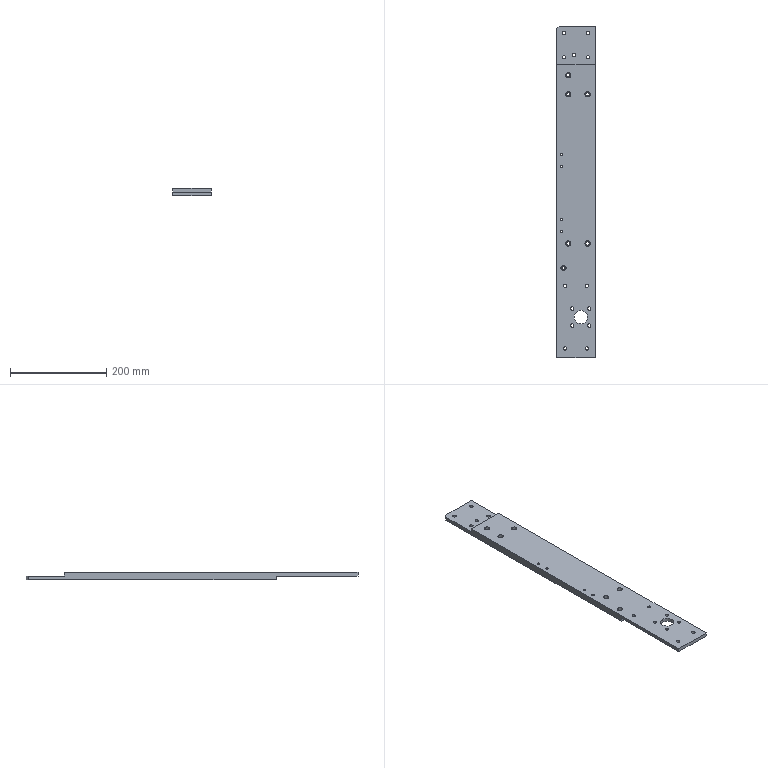Component | SolidWorks | VerticalPlate(1)-1 | 1 solid | 85 faces | volume 663200 mm3 | cylinder 60 | plane 17 | cone 8 | commonest cylinder face diameters 7 x38 11 x12 4.2 x8 28 x2